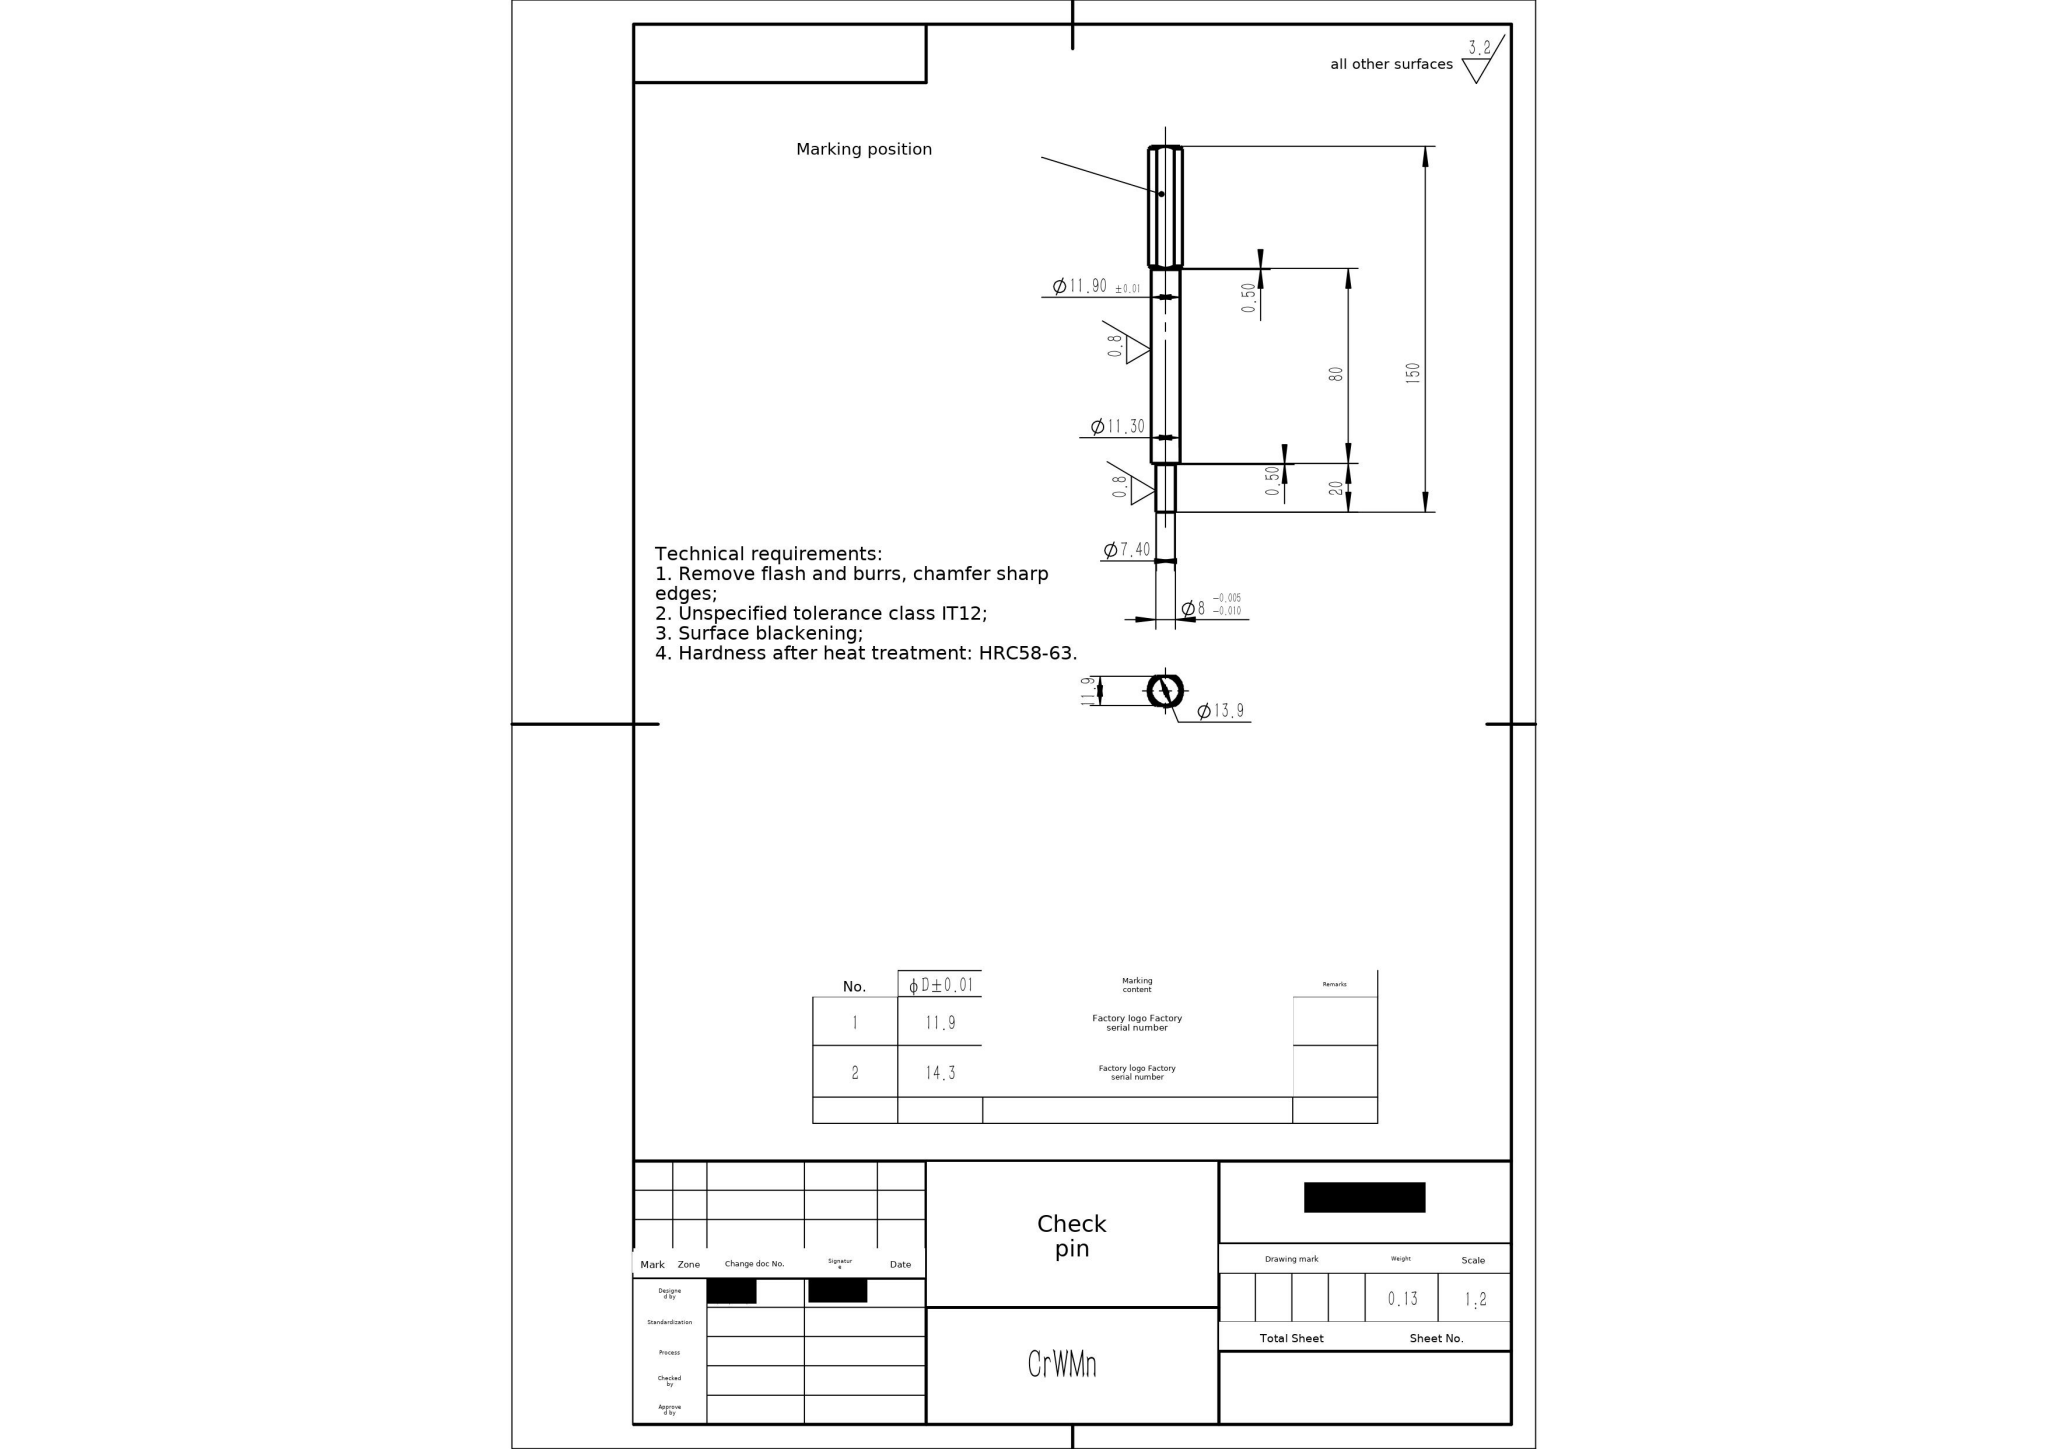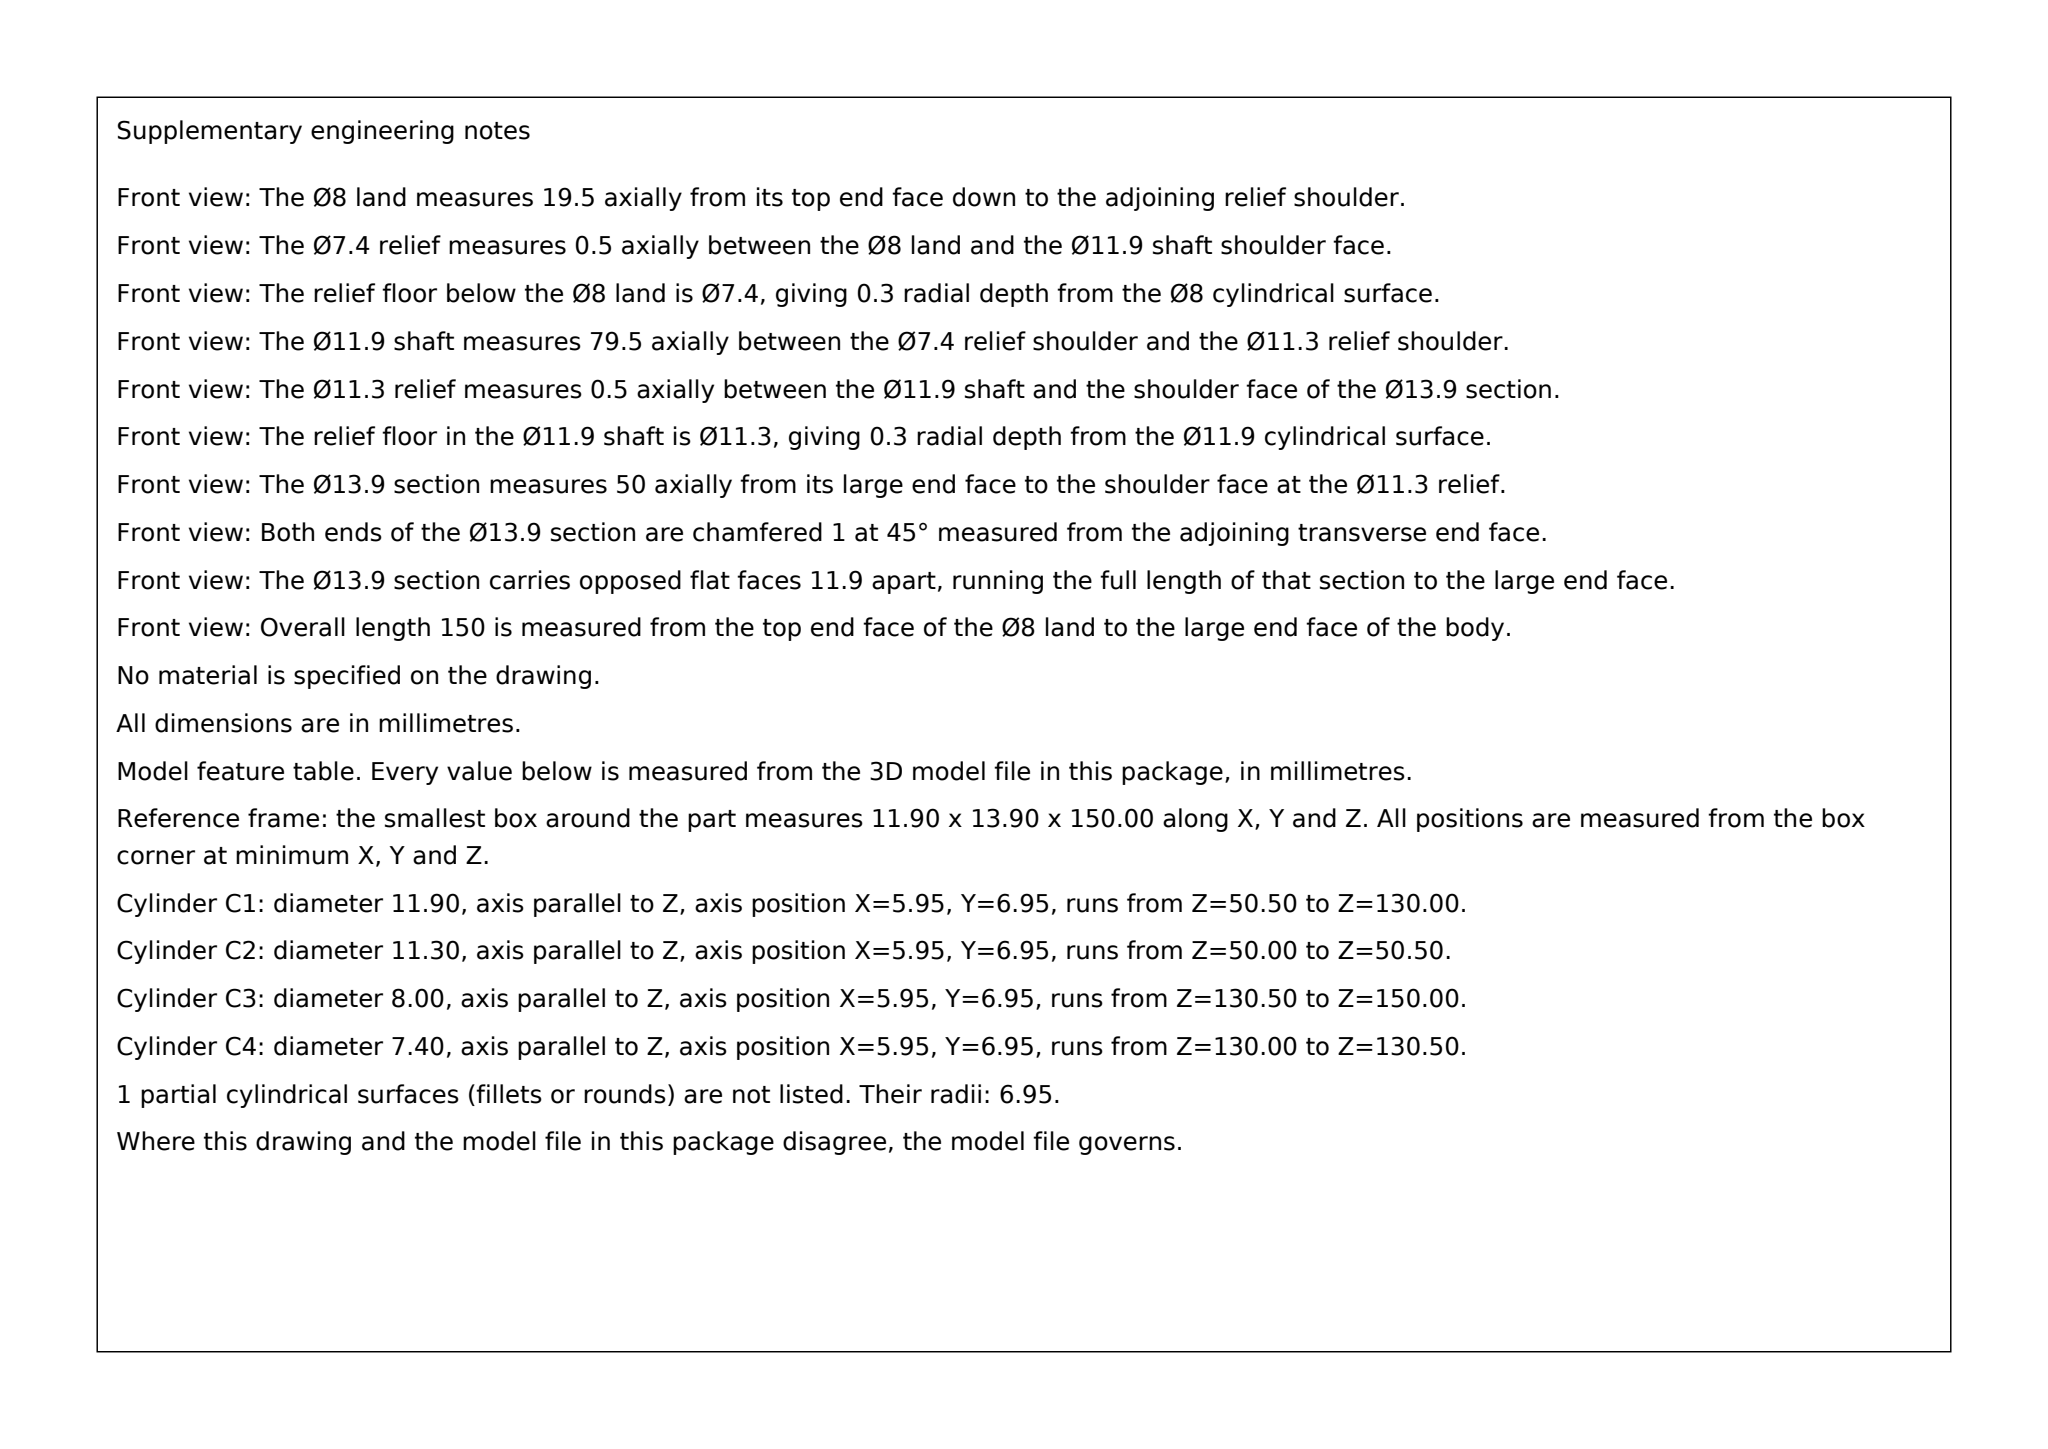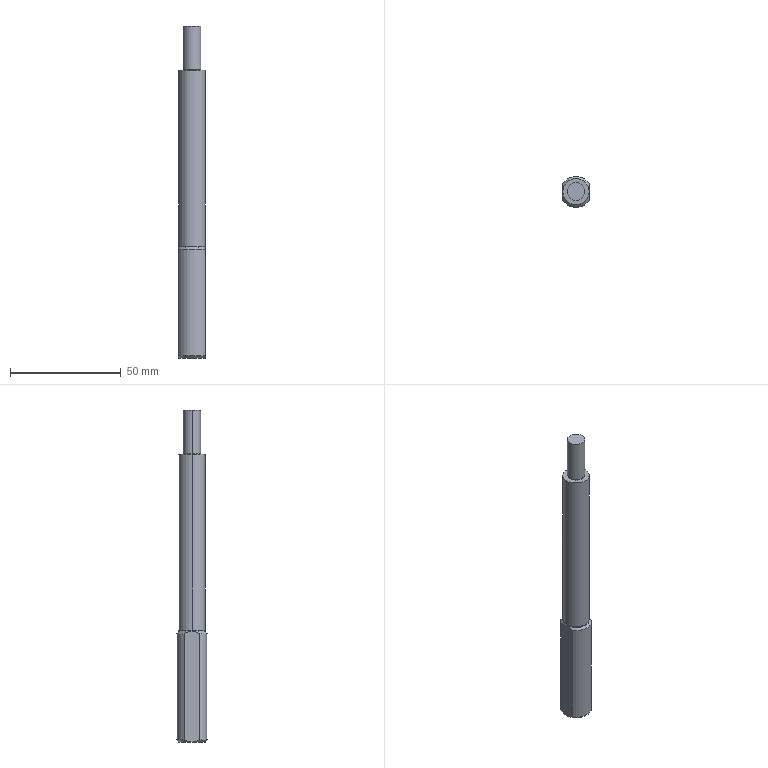Part | SolidWorks | mm | 1 solid | 22 faces | box 11.9 x 13.9 x 150 mm | volume 16965 mm3 | cylinder 10 | plane 8 | cone 4 | commonest cylinder face diameters 11.3 x2 8 x2 7.4 x2 11.9 x2 13.9 x2
Drawing notes:
2X FLAT ON Ø13.9 HEAD: 11.9 A/F x 50 LG FROM HEAD END FACE | from the solid: x-normal planes at 1.0 and 12.9 (ctr 6.95) = 11.9 across flats on Ø13.9 head; head region bounded by z-planes 0 and 50 (48 cyl + 2X C1)
45° TRANSITION BOTH ENDS Ø11.90 SHAFT, TO Ø11.30 AND TO Ø7.40 | from the solid: cones[90.0, ref_dia 11.9] count 2 at the ends of the Ø11.9 x 79.5 cylinder (z 50.5 and 130), adjoining Ø11.3 and Ø7.4 x 0.5 reliefs
STEP:
#1=CARTESIAN_POINT('',(5.65,0.,-80.));
#2=VERTEX_POINT('',#1);
#3=CARTESIAN_POINT('',(-5.65,0.,-80.));
#4=VERTEX_POINT('',#3);
#5=CARTESIAN_POINT('',(0.,0.,-80.));
#6=DIRECTION('',(0.,0.,1.));
#7=DIRECTION('',(1.,0.,0.));
#8=AXIS2_PLACEMENT_3D('',#5,#6,#7);
#9=CIRCLE('',#8,5.65);
#10=EDGE_CURVE('',#2,#4,#9,.T.);
#11=ORIENTED_EDGE('',*,*,#10,.T.);
#12=CARTESIAN_POINT('',(-5.65,0.,-79.5));
#13=VERTEX_POINT('',#12);
#14=CARTESIAN_POINT('',(-5.65,0.,20.));
#15=DIRECTION('',(0.,0.,1.));
#16=VECTOR('',#15,1000.);
#17=LINE('',#14,#16);
#18=EDGE_CURVE('',#4,#13,#17,.T.);
#19=ORIENTED_EDGE('',*,*,#18,.T.);
#20=CARTESIAN_POINT('',(5.65,0.,-79.5));
#21=VERTEX_POINT('',#20);
#22=CARTESIAN_POINT('',(0.,0.,-79.5));
#23=DIRECTION('',(0.,0.,1.));
#24=DIRECTION('',(1.,0.,0.));
#25=AXIS2_PLACEMENT_3D('',#22,#23,#24);
#26=CIRCLE('',#25,5.65);
#27=EDGE_CURVE('',#21,#13,#26,.T.);
#28=ORIENTED_EDGE('',*,*,#27,.F.);
#29=CARTESIAN_POINT('',(5.65,0.,20.));
#30=DIRECTION('',(0.,0.,1.));
#31=VECTOR('',#30,1000.);
#32=LINE('',#29,#31);
#33=EDGE_CURVE('',#2,#21,#32,.T.);
#34=ORIENTED_EDGE('',*,*,#33,.F.);
#35=EDGE_LOOP('',(#11,#19,#28,#34));
#36=FACE_OUTER_BOUND('',#35,.T.);
#37=CARTESIAN_POINT('',(0.,0.,20.));
#38=DIRECTION('',(0.,0.,1.));
#39=DIRECTION('',(1.,0.,0.));
#40=AXIS2_PLACEMENT_3D('',#37,#38,#39);
#41=CYLINDRICAL_SURFACE('',#40,5.65);
#42=ADVANCED_FACE('',(#36),#41,.T.);
#43=CARTESIAN_POINT('',(4.,0.,20.));
#44=VERTEX_POINT('',#43);
#45=CARTESIAN_POINT('',(-4.,0.,20.));
#46=VERTEX_POINT('',#45);
#47=CARTESIAN_POINT('',(0.,0.,20.));
#48=DIRECTION('',(0.,0.,1.));
#49=DIRECTION('',(1.,0.,0.));
#50=AXIS2_PLACEMENT_3D('',#47,#48,#49);
#51=CIRCLE('',#50,4.);
#52=EDGE_CURVE('',#44,#46,#51,.T.);
#53=ORIENTED_EDGE('',*,*,#52,.F.);
#54=CARTESIAN_POINT('',(4.,0.,0.5));
#55=VERTEX_POINT('',#54);
#56=CARTESIAN_POINT('',(4.,0.,20.));
#57=DIRECTION('',(0.,0.,-1.));
#58=VECTOR('',#57,1000.);
#59=LINE('',#56,#58);
#60=EDGE_CURVE('',#44,#55,#59,.T.);
#61=ORIENTED_EDGE('',*,*,#60,.T.);
#62=CARTESIAN_POINT('',(-4.,0.,0.5));
#63=VERTEX_POINT('',#62);
#64=CARTESIAN_POINT('',(0.,0.,0.5));
#65=DIRECTION('',(0.,0.,1.));
#66=DIRECTION('',(1.,0.,0.));
#67=AXIS2_PLACEMENT_3D('',#64,#65,#66);
#68=CIRCLE('',#67,4.);
#69=EDGE_CURVE('',#55,#63,#68,.T.);
#70=ORIENTED_EDGE('',*,*,#69,.T.);
#71=CARTESIAN_POINT('',(-4.,0.,20.));
#72=DIRECTION('',(0.,0.,-1.));
#73=VECTOR('',#72,1000.);
#74=LINE('',#71,#73);
#75=EDGE_CURVE('',#46,#63,#74,.T.);
#76=ORIENTED_EDGE('',*,*,#75,.F.);
#77=EDGE_LOOP('',(#53,#61,#70,#76));
#78=FACE_OUTER_BOUND('',#77,.T.);
#79=CARTESIAN_POINT('',(0.,0.,20.));
#80=DIRECTION('',(0.,0.,-1.));
#81=DIRECTION('',(-1.,0.,0.));
#82=AXIS2_PLACEMENT_3D('',#79,#80,#81);
#83=CYLINDRICAL_SURFACE('',#82,4.);
#84=ADVANCED_FACE('',(#78),#83,.T.);
#85=CARTESIAN_POINT('',(3.7,0.,0.));
#86=VERTEX_POINT('',#85);
#87=CARTESIAN_POINT('',(-3.7,0.,0.));
#88=VERTEX_POINT('',#87);
#89=CARTESIAN_POINT('',(0.,0.,0.));
#90=DIRECTION('',(0.,0.,1.));
#91=DIRECTION('',(1.,0.,0.));
#92=AXIS2_PLACEMENT_3D('',#89,#90,#91);
#93=CIRCLE('',#92,3.7);
#94=EDGE_CURVE('',#86,#88,#93,.T.);
#95=ORIENTED_EDGE('',*,*,#94,.T.);
#96=CARTESIAN_POINT('',(-3.7,0.,0.5));
#97=VERTEX_POINT('',#96);
#98=CARTESIAN_POINT('',(-3.7,0.,20.));
#99=DIRECTION('',(0.,0.,1.));
#100=VECTOR('',#99,1000.);
#101=LINE('',#98,#100);
#102=EDGE_CURVE('',#88,#97,#101,.T.);
#103=ORIENTED_EDGE('',*,*,#102,.T.);
#104=CARTESIAN_POINT('',(3.7,0.,0.5));
#105=VERTEX_POINT('',#104);
#106=CARTESIAN_POINT('',(0.,0.,0.5));
#107=DIRECTION('',(0.,0.,1.));
#108=DIRECTION('',(1.,0.,0.));
#109=AXIS2_PLACEMENT_3D('',#106,#107,#108);
#110=CIRCLE('',#109,3.7);
#111=EDGE_CURVE('',#105,#97,#110,.T.);
#112=ORIENTED_EDGE('',*,*,#111,.F.);
#113=CARTESIAN_POINT('',(3.7,0.,20.));
#114=DIRECTION('',(0.,0.,1.));
#115=VECTOR('',#114,1000.);
#116=LINE('',#113,#115);
#117=EDGE_CURVE('',#86,#105,#116,.T.);
#118=ORIENTED_EDGE('',*,*,#117,.F.);
#119=EDGE_LOOP('',(#95,#103,#112,#118));
#120=FACE_OUTER_BOUND('',#119,.T.);
#121=CARTESIAN_POINT('',(0.,0.,20.));
#122=DIRECTION('',(0.,0.,1.));
#123=DIRECTION('',(1.,0.,0.));
#124=AXIS2_PLACEMENT_3D('',#121,#122,#123);
#125=CYLINDRICAL_SURFACE('',#124,3.7);
#126=ADVANCED_FACE('',(#120),#125,.T.);
#127=CARTESIAN_POINT('',(5.95,0.,-79.5));
#128=VERTEX_POINT('',#127);
#129=CARTESIAN_POINT('',(-5.95,0.,-79.5));
#130=VERTEX_POINT('',#129);
#131=CARTESIAN_POINT('',(0.,0.,-79.5));
#132=DIRECTION('',(0.,0.,1.));
#133=DIRECTION('',(1.,0.,0.));
#134=AXIS2_PLACEMENT_3D('',#131,#132,#133);
#135=CIRCLE('',#134,5.95);
#136=EDGE_CURVE('',#128,#130,#135,.T.);
#137=ORIENTED_EDGE('',*,*,#136,.T.);
#138=CARTESIAN_POINT('',(-5.95,0.,0.));
#139=VERTEX_POINT('',#138);
#140=CARTESIAN_POINT('',(-5.95,0.,-80.));
#141=DIRECTION('',(0.,0.,1.));
#142=VECTOR('',#141,1000.);
#143=LINE('',#140,#142);
#144=EDGE_CURVE('',#130,#139,#143,.T.);
#145=ORIENTED_EDGE('',*,*,#144,.T.);
#146=CARTESIAN_POINT('',(5.95,0.,0.));
#147=VERTEX_POINT('',#146);
#148=CARTESIAN_POINT('',(0.,0.,0.));
#149=DIRECTION('',(0.,0.,-1.));
#150=DIRECTION('',(-1.,0.,0.));
#151=AXIS2_PLACEMENT_3D('',#148,#149,#150);
#152=CIRCLE('',#151,5.95);
#153=EDGE_CURVE('',#139,#147,#152,.T.);
#154=ORIENTED_EDGE('',*,*,#153,.T.);
#155=CARTESIAN_POINT('',(5.95,0.,-80.));
#156=DIRECTION('',(0.,0.,1.));
#157=VECTOR('',#156,1000.);
#158=LINE('',#155,#157);
#159=EDGE_CURVE('',#128,#147,#158,.T.);
#160=ORIENTED_EDGE('',*,*,#159,.F.);
#161=EDGE_LOOP('',(#137,#145,#154,#160));
#162=FACE_OUTER_BOUND('',#161,.T.);
#163=CARTESIAN_POINT('',(0.,0.,-80.));
#164=DIRECTION('',(0.,0.,1.));
#165=DIRECTION('',(1.,0.,0.));
#166=AXIS2_PLACEMENT_3D('',#163,#164,#165);
#167=CYLINDRICAL_SURFACE('',#166,5.95);
#168=ADVANCED_FACE('',(#162),#167,.T.);
#169=ORIENTED_EDGE('',*,*,#144,.F.);
#170=CARTESIAN_POINT('',(0.,0.,-79.5));
#171=DIRECTION('',(0.,0.,1.));
#172=DIRECTION('',(1.,0.,0.));
#173=AXIS2_PLACEMENT_3D('',#170,#171,#172);
#174=CIRCLE('',#173,5.95);
#175=EDGE_CURVE('',#130,#128,#174,.T.);
#176=ORIENTED_EDGE('',*,*,#175,.T.);
#177=ORIENTED_EDGE('',*,*,#159,.T.);
#178=CARTESIAN_POINT('',(0.,0.,0.));
#179=DIRECTION('',(0.,0.,-1.));
#180=DIRECTION('',(-1.,0.,0.));
#181=AXIS2_PLACEMENT_3D('',#178,#179,#180);
#182=CIRCLE('',#181,5.95);
#183=EDGE_CURVE('',#147,#139,#182,.T.);
#184=ORIENTED_EDGE('',*,*,#183,.T.);
#185=EDGE_LOOP('',(#169,#176,#177,#184));
#186=FACE_OUTER_BOUND('',#185,.T.);
#187=CARTESIAN_POINT('',(0.,0.,-80.));
#188=DIRECTION('',(0.,0.,1.));
#189=DIRECTION('',(1.,0.,0.));
#190=AXIS2_PLACEMENT_3D('',#187,#188,#189);
#191=CYLINDRICAL_SURFACE('',#190,5.95);
#192=ADVANCED_FACE('',(#186),#191,.T.);
#193=ORIENTED_EDGE('',*,*,#183,.F.);
#194=ORIENTED_EDGE('',*,*,#153,.F.);
#195=EDGE_LOOP('',(#193,#194));
#196=FACE_OUTER_BOUND('',#195,.T.);
#197=ORIENTED_EDGE('',*,*,#94,.F.);
#198=CARTESIAN_POINT('',(0.,0.,0.));
#199=DIRECTION('',(0.,0.,1.));
#200=DIRECTION('',(1.,0.,0.));
#201=AXIS2_PLACEMENT_3D('',#198,#199,#200);
#202=CIRCLE('',#201,3.7);
#203=EDGE_CURVE('',#88,#86,#202,.T.);
#204=ORIENTED_EDGE('',*,*,#203,.F.);
#205=EDGE_LOOP('',(#197,#204));
#206=FACE_BOUND('',#205,.T.);
#207=CARTESIAN_POINT('',(0.,0.,0.));
#208=DIRECTION('',(0.,0.,-1.));
#209=DIRECTION('',(-1.,0.,0.));
#210=AXIS2_PLACEMENT_3D('',#207,#208,#209);
#211=PLANE('',#210);
#212=ADVANCED_FACE('',(#196,#206),#211,.F.);
#213=ORIENTED_EDGE('',*,*,#102,.F.);
#214=ORIENTED_EDGE('',*,*,#203,.T.);
#215=ORIENTED_EDGE('',*,*,#117,.T.);
#216=CARTESIAN_POINT('',(0.,0.,0.5));
#217=DIRECTION('',(0.,0.,1.));
#218=DIRECTION('',(1.,0.,0.));
#219=AXIS2_PLACEMENT_3D('',#216,#217,#218);
#220=CIRCLE('',#219,3.7);
#221=EDGE_CURVE('',#97,#105,#220,.T.);
#222=ORIENTED_EDGE('',*,*,#221,.F.);
#223=EDGE_LOOP('',(#213,#214,#215,#222));
#224=FACE_OUTER_BOUND('',#223,.T.);
#225=CARTESIAN_POINT('',(0.,0.,20.));
#226=DIRECTION('',(0.,0.,1.));
#227=DIRECTION('',(1.,0.,0.));
#228=AXIS2_PLACEMENT_3D('',#225,#226,#227);
#229=CYLINDRICAL_SURFACE('',#228,3.7);
#230=ADVANCED_FACE('',(#224),#229,.T.);
#231=ORIENTED_EDGE('',*,*,#111,.T.);
#232=ORIENTED_EDGE('',*,*,#221,.T.);
#233=EDGE_LOOP('',(#231,#232));
#234=FACE_BOUND('',#233,.T.);
#235=CARTESIAN_POINT('',(0.,0.,0.5));
#236=DIRECTION('',(0.,0.,1.));
#237=DIRECTION('',(1.,0.,0.));
#238=AXIS2_PLACEMENT_3D('',#235,#236,#237);
#239=CIRCLE('',#238,4.);
#240=EDGE_CURVE('',#63,#55,#239,.T.);
#241=ORIENTED_EDGE('',*,*,#240,.F.);
#242=ORIENTED_EDGE('',*,*,#69,.F.);
#243=EDGE_LOOP('',(#241,#242));
#244=FACE_OUTER_BOUND('',#243,.T.);
#245=CARTESIAN_POINT('',(0.,4.,0.5));
#246=DIRECTION('',(0.,0.,-1.));
#247=DIRECTION('',(-1.,0.,0.));
#248=AXIS2_PLACEMENT_3D('',#245,#246,#247);
#249=PLANE('',#248);
#250=ADVANCED_FACE('',(#234,#244),#249,.T.);
#251=CARTESIAN_POINT('',(0.,0.,20.));
#252=DIRECTION('',(0.,0.,1.));
#253=DIRECTION('',(1.,0.,0.));
#254=AXIS2_PLACEMENT_3D('',#251,#252,#253);
#255=CIRCLE('',#254,4.);
#256=EDGE_CURVE('',#46,#44,#255,.T.);
#257=ORIENTED_EDGE('',*,*,#256,.T.);
#258=ORIENTED_EDGE('',*,*,#52,.T.);
#259=EDGE_LOOP('',(#257,#258));
#260=FACE_OUTER_BOUND('',#259,.T.);
#261=CARTESIAN_POINT('',(0.,0.,20.));
#262=DIRECTION('',(0.,0.,1.));
#263=DIRECTION('',(1.,0.,0.));
#264=AXIS2_PLACEMENT_3D('',#261,#262,#263);
#265=PLANE('',#264);
#266=ADVANCED_FACE('',(#260),#265,.T.);
#267=ORIENTED_EDGE('',*,*,#60,.F.);
#268=ORIENTED_EDGE('',*,*,#256,.F.);
#269=ORIENTED_EDGE('',*,*,#75,.T.);
#270=ORIENTED_EDGE('',*,*,#240,.T.);
#271=EDGE_LOOP('',(#267,#268,#269,#270));
#272=FACE_OUTER_BOUND('',#271,.T.);
#273=CARTESIAN_POINT('',(0.,0.,20.));
#274=DIRECTION('',(0.,0.,-1.));
#275=DIRECTION('',(-1.,0.,0.));
#276=AXIS2_PLACEMENT_3D('',#273,#274,#275);
#277=CYLINDRICAL_SURFACE('',#276,4.);
#278=ADVANCED_FACE('',(#272),#277,.T.);
#279=ORIENTED_EDGE('',*,*,#18,.F.);
#280=CARTESIAN_POINT('',(0.,0.,-80.));
#281=DIRECTION('',(0.,0.,1.));
#282=DIRECTION('',(1.,0.,0.));
#283=AXIS2_PLACEMENT_3D('',#280,#281,#282);
#284=CIRCLE('',#283,5.65);
#285=EDGE_CURVE('',#4,#2,#284,.T.);
#286=ORIENTED_EDGE('',*,*,#285,.T.);
#287=ORIENTED_EDGE('',*,*,#33,.T.);
#288=CARTESIAN_POINT('',(0.,0.,-79.5));
#289=DIRECTION('',(0.,0.,1.));
#290=DIRECTION('',(1.,0.,0.));
#291=AXIS2_PLACEMENT_3D('',#288,#289,#290);
#292=CIRCLE('',#291,5.65);
#293=EDGE_CURVE('',#13,#21,#292,.T.);
#294=ORIENTED_EDGE('',*,*,#293,.F.);
#295=EDGE_LOOP('',(#279,#286,#287,#294));
#296=FACE_OUTER_BOUND('',#295,.T.);
#297=CARTESIAN_POINT('',(0.,0.,20.));
#298=DIRECTION('',(0.,0.,1.));
#299=DIRECTION('',(1.,0.,0.));
#300=AXIS2_PLACEMENT_3D('',#297,#298,#299);
#301=CYLINDRICAL_SURFACE('',#300,5.65);
#302=ADVANCED_FACE('',(#296),#301,.T.);
#303=ORIENTED_EDGE('',*,*,#27,.T.);
#304=ORIENTED_EDGE('',*,*,#293,.T.);
#305=EDGE_LOOP('',(#303,#304));
#306=FACE_BOUND('',#305,.T.);
#307=ORIENTED_EDGE('',*,*,#136,.F.);
#308=ORIENTED_EDGE('',*,*,#175,.F.);
#309=EDGE_LOOP('',(#307,#308));
#310=FACE_OUTER_BOUND('',#309,.T.);
#311=CARTESIAN_POINT('',(0.,5.95,-79.5));
#312=DIRECTION('',(0.,0.,-1.));
#313=DIRECTION('',(-1.,0.,0.));
#314=AXIS2_PLACEMENT_3D('',#311,#312,#313);
#315=PLANE('',#314);
#316=ADVANCED_FACE('',(#306,#310),#315,.T.);
#317=CARTESIAN_POINT('',(-5.95,0.,-130.));
#318=VERTEX_POINT('',#317);
#319=CARTESIAN_POINT('',(5.95,0.,-130.));
#320=VERTEX_POINT('',#319);
#321=CARTESIAN_POINT('',(0.,0.,-130.));
#322=DIRECTION('',(0.,0.,-1.));
#323=DIRECTION('',(-1.,0.,0.));
#324=AXIS2_PLACEMENT_3D('',#321,#322,#323);
#325=CIRCLE('',#324,5.95);
#326=EDGE_CURVE('',#318,#320,#325,.T.);
#327=ORIENTED_EDGE('',*,*,#326,.T.);
#328=CARTESIAN_POINT('',(0.,0.,-130.));
#329=DIRECTION('',(0.,0.,-1.));
#330=DIRECTION('',(-1.,0.,0.));
#331=AXIS2_PLACEMENT_3D('',#328,#329,#330);
#332=CIRCLE('',#331,5.95);
#333=EDGE_CURVE('',#320,#318,#332,.T.);
#334=ORIENTED_EDGE('',*,*,#333,.T.);
#335=EDGE_LOOP('',(#327,#334));
#336=FACE_OUTER_BOUND('',#335,.T.);
#337=CARTESIAN_POINT('',(0.,0.,-130.));
#338=DIRECTION('',(0.,0.,-1.));
#339=DIRECTION('',(-1.,0.,0.));
#340=AXIS2_PLACEMENT_3D('',#337,#338,#339);
#341=PLANE('',#340);
#342=ADVANCED_FACE('',(#336),#341,.T.);
#343=CARTESIAN_POINT('',(5.95,3.592,-129.));
#344=VERTEX_POINT('',#343);
#345=CARTESIAN_POINT('',(5.95,3.592,-81.));
#346=VERTEX_POINT('',#345);
#347=CARTESIAN_POINT('',(5.95,3.592,-130.));
#348=DIRECTION('',(0.,0.,1.));
#349=VECTOR('',#348,1000.);
#350=LINE('',#347,#349);
#351=EDGE_CURVE('',#344,#346,#350,.T.);
#352=ORIENTED_EDGE('',*,*,#351,.F.);
#353=CARTESIAN_POINT('',(-5.95,3.592,-129.));
#354=VERTEX_POINT('',#353);
#355=CARTESIAN_POINT('',(0.,0.,-129.));
#356=DIRECTION('',(0.,0.,1.));
#357=DIRECTION('',(-1.,-0.,0.));
#358=AXIS2_PLACEMENT_3D('',#355,#356,#357);
#359=CIRCLE('',#358,6.95);
#360=EDGE_CURVE('',#344,#354,#359,.T.);
#361=ORIENTED_EDGE('',*,*,#360,.T.);
#362=CARTESIAN_POINT('',(-5.95,3.592,-81.));
#363=VERTEX_POINT('',#362);
#364=CARTESIAN_POINT('',(-5.95,3.592,-130.));
#365=DIRECTION('',(0.,0.,1.));
#366=VECTOR('',#365,1000.);
#367=LINE('',#364,#366);
#368=EDGE_CURVE('',#354,#363,#367,.T.);
#369=ORIENTED_EDGE('',*,*,#368,.T.);
#370=CARTESIAN_POINT('',(0.,0.,-81.));
#371=DIRECTION('',(0.,0.,-1.));
#372=DIRECTION('',(-1.,0.,0.));
#373=AXIS2_PLACEMENT_3D('',#370,#371,#372);
#374=CIRCLE('',#373,6.95);
#375=EDGE_CURVE('',#363,#346,#374,.T.);
#376=ORIENTED_EDGE('',*,*,#375,.T.);
#377=EDGE_LOOP('',(#352,#361,#369,#376));
#378=FACE_OUTER_BOUND('',#377,.T.);
#379=CARTESIAN_POINT('',(0.,0.,-130.));
#380=DIRECTION('',(0.,0.,1.));
#381=DIRECTION('',(1.,0.,0.));
#382=AXIS2_PLACEMENT_3D('',#379,#380,#381);
#383=CYLINDRICAL_SURFACE('',#382,6.95);
#384=ADVANCED_FACE('',(#378),#383,.T.);
#385=CARTESIAN_POINT('',(-5.95,-3.592,-81.));
#386=VERTEX_POINT('',#385);
#387=CARTESIAN_POINT('',(-5.95,-3.592,-129.));
#388=VERTEX_POINT('',#387);
#389=CARTESIAN_POINT('',(-5.95,-3.592,-130.));
#390=DIRECTION('',(0.,0.,-1.));
#391=VECTOR('',#390,1000.);
#392=LINE('',#389,#391);
#393=EDGE_CURVE('',#386,#388,#392,.T.);
#394=ORIENTED_EDGE('',*,*,#393,.T.);
#395=CARTESIAN_POINT('',(5.95,-3.592,-129.));
#396=VERTEX_POINT('',#395);
#397=CARTESIAN_POINT('',(0.,0.,-129.));
#398=DIRECTION('',(0.,0.,1.));
#399=DIRECTION('',(-1.,0.,0.));
#400=AXIS2_PLACEMENT_3D('',#397,#398,#399);
#401=CIRCLE('',#400,6.95);
#402=EDGE_CURVE('',#388,#396,#401,.T.);
#403=ORIENTED_EDGE('',*,*,#402,.T.);
#404=CARTESIAN_POINT('',(5.95,-3.592,-81.));
#405=VERTEX_POINT('',#404);
#406=CARTESIAN_POINT('',(5.95,-3.592,-130.));
#407=DIRECTION('',(0.,0.,-1.));
#408=VECTOR('',#407,1000.);
#409=LINE('',#406,#408);
#410=EDGE_CURVE('',#405,#396,#409,.T.);
#411=ORIENTED_EDGE('',*,*,#410,.F.);
#412=CARTESIAN_POINT('',(0.,0.,-81.));
#413=DIRECTION('',(0.,0.,-1.));
#414=DIRECTION('',(-1.,0.,0.));
#415=AXIS2_PLACEMENT_3D('',#412,#413,#414);
#416=CIRCLE('',#415,6.95);
#417=EDGE_CURVE('',#405,#386,#416,.T.);
#418=ORIENTED_EDGE('',*,*,#417,.T.);
#419=EDGE_LOOP('',(#394,#403,#411,#418));
#420=FACE_OUTER_BOUND('',#419,.T.);
#421=CARTESIAN_POINT('',(0.,0.,-130.));
#422=DIRECTION('',(0.,0.,1.));
#423=DIRECTION('',(1.,0.,0.));
#424=AXIS2_PLACEMENT_3D('',#421,#422,#423);
#425=CYLINDRICAL_SURFACE('',#424,6.95);
#426=ADVANCED_FACE('',(#420),#425,.T.);
#427=CARTESIAN_POINT('',(-5.95,3.592,-129.));
#428=CARTESIAN_POINT('',(-5.95,3.033,-129.289));
#429=CARTESIAN_POINT('',(-5.95,2.459,-129.537));
#430=CARTESIAN_POINT('',(-5.95,1.263,-129.894));
#431=CARTESIAN_POINT('',(-5.95,0.6334,-130.));
#432=CARTESIAN_POINT('',(-5.95,0.,-130.));
#433=B_SPLINE_CURVE_WITH_KNOTS('',3,(#427,#428,#429,#430,#431,#432),.UNSPECIFIED.,.F.,.F.,(4,2,4),(0.,0.00187,0.00374),.UNSPECIFIED.);
#434=EDGE_CURVE('',#354,#318,#433,.T.);
#435=ORIENTED_EDGE('',*,*,#434,.T.);
#436=CARTESIAN_POINT('',(-5.95,0.,-130.));
#437=CARTESIAN_POINT('',(-5.95,-0.6327,-130.));
#438=CARTESIAN_POINT('',(-5.95,-1.248,-129.898));
#439=CARTESIAN_POINT('',(-5.95,-2.15,-129.63));
#440=CARTESIAN_POINT('',(-5.95,-2.447,-129.522));
#441=CARTESIAN_POINT('',(-5.95,-3.027,-129.279));
#442=CARTESIAN_POINT('',(-5.95,-3.312,-129.145));
#443=CARTESIAN_POINT('',(-5.95,-3.592,-129.));
#444=B_SPLINE_CURVE_WITH_KNOTS('',3,(#436,#437,#438,#439,#440,#441,#442,#443),.UNSPECIFIED.,.F.,.F.,(4,2,2,4),(0.,0.00187,0.002805,0.00374),.UNSPECIFIED.);
#445=EDGE_CURVE('',#318,#388,#444,.T.);
#446=ORIENTED_EDGE('',*,*,#445,.T.);
#447=ORIENTED_EDGE('',*,*,#393,.F.);
#448=CARTESIAN_POINT('',(-5.95,-0.,-80.));
#449=VERTEX_POINT('',#448);
#450=CARTESIAN_POINT('',(-5.95,-3.592,-81.));
#451=CARTESIAN_POINT('',(-5.95,-3.033,-80.711));
#452=CARTESIAN_POINT('',(-5.95,-2.459,-80.463));
#453=CARTESIAN_POINT('',(-5.95,-1.263,-80.106));
#454=CARTESIAN_POINT('',(-5.95,-0.6334,-80.));
#455=CARTESIAN_POINT('',(-5.95,-0.,-80.));
#456=B_SPLINE_CURVE_WITH_KNOTS('',3,(#450,#451,#452,#453,#454,#455),.UNSPECIFIED.,.F.,.F.,(4,2,4),(0.,0.00187,0.00374),.UNSPECIFIED.);
#457=EDGE_CURVE('',#386,#449,#456,.T.);
#458=ORIENTED_EDGE('',*,*,#457,.T.);
#459=CARTESIAN_POINT('',(-5.95,-0.,-80.));
#460=CARTESIAN_POINT('',(-5.95,0.6327,-80.));
#461=CARTESIAN_POINT('',(-5.95,1.248,-80.102));
#462=CARTESIAN_POINT('',(-5.95,2.15,-80.37));
#463=CARTESIAN_POINT('',(-5.95,2.447,-80.478));
#464=CARTESIAN_POINT('',(-5.95,3.027,-80.721));
#465=CARTESIAN_POINT('',(-5.95,3.312,-80.855));
#466=CARTESIAN_POINT('',(-5.95,3.592,-81.));
#467=B_SPLINE_CURVE_WITH_KNOTS('',3,(#459,#460,#461,#462,#463,#464,#465,#466),.UNSPECIFIED.,.F.,.F.,(4,2,2,4),(0.,0.00187,0.002805,0.00374),.UNSPECIFIED.);
#468=EDGE_CURVE('',#449,#363,#467,.T.);
#469=ORIENTED_EDGE('',*,*,#468,.T.);
#470=ORIENTED_EDGE('',*,*,#368,.F.);
#471=EDGE_LOOP('',(#435,#446,#447,#458,#469,#470));
#472=FACE_OUTER_BOUND('',#471,.T.);
#473=CARTESIAN_POINT('',(-5.95,15.,-130.));
#474=DIRECTION('',(1.,0.,0.));
#475=DIRECTION('',(-0.,1.,0.));
#476=AXIS2_PLACEMENT_3D('',#473,#474,#475);
#477=PLANE('',#476);
#478=ADVANCED_FACE('',(#472),#477,.F.);
#479=ORIENTED_EDGE('',*,*,#410,.T.);
#480=CARTESIAN_POINT('',(5.95,-3.592,-129.));
#481=CARTESIAN_POINT('',(5.95,-3.033,-129.289));
#482=CARTESIAN_POINT('',(5.95,-2.459,-129.537));
#483=CARTESIAN_POINT('',(5.95,-1.263,-129.894));
#484=CARTESIAN_POINT('',(5.95,-0.6334,-130.));
#485=CARTESIAN_POINT('',(5.95,0.,-130.));
#486=B_SPLINE_CURVE_WITH_KNOTS('',3,(#480,#481,#482,#483,#484,#485),.UNSPECIFIED.,.F.,.F.,(4,2,4),(0.,0.00187,0.00374),.UNSPECIFIED.);
#487=EDGE_CURVE('',#396,#320,#486,.T.);
#488=ORIENTED_EDGE('',*,*,#487,.T.);
#489=CARTESIAN_POINT('',(5.95,0.,-130.));
#490=CARTESIAN_POINT('',(5.95,0.6327,-130.));
#491=CARTESIAN_POINT('',(5.95,1.248,-129.898));
#492=CARTESIAN_POINT('',(5.95,2.15,-129.63));
#493=CARTESIAN_POINT('',(5.95,2.447,-129.522));
#494=CARTESIAN_POINT('',(5.95,3.027,-129.279));
#495=CARTESIAN_POINT('',(5.95,3.312,-129.145));
#496=CARTESIAN_POINT('',(5.95,3.592,-129.));
#497=B_SPLINE_CURVE_WITH_KNOTS('',3,(#489,#490,#491,#492,#493,#494,#495,#496),.UNSPECIFIED.,.F.,.F.,(4,2,2,4),(0.,0.00187,0.002805,0.00374),.UNSPECIFIED.);
#498=EDGE_CURVE('',#320,#344,#497,.T.);
#499=ORIENTED_EDGE('',*,*,#498,.T.);
#500=ORIENTED_EDGE('',*,*,#351,.T.);
#501=CARTESIAN_POINT('',(5.95,-0.,-80.));
#502=VERTEX_POINT('',#501);
#503=CARTESIAN_POINT('',(5.95,3.592,-81.));
#504=CARTESIAN_POINT('',(5.95,3.033,-80.711));
#505=CARTESIAN_POINT('',(5.95,2.459,-80.463));
#506=CARTESIAN_POINT('',(5.95,1.263,-80.106));
#507=CARTESIAN_POINT('',(5.95,0.6334,-80.));
#508=CARTESIAN_POINT('',(5.95,-0.,-80.));
#509=B_SPLINE_CURVE_WITH_KNOTS('',3,(#503,#504,#505,#506,#507,#508),.UNSPECIFIED.,.F.,.F.,(4,2,4),(0.,0.00187,0.00374),.UNSPECIFIED.);
#510=EDGE_CURVE('',#346,#502,#509,.T.);
#511=ORIENTED_EDGE('',*,*,#510,.T.);
#512=CARTESIAN_POINT('',(5.95,-0.,-80.));
#513=CARTESIAN_POINT('',(5.95,-0.6327,-80.));
#514=CARTESIAN_POINT('',(5.95,-1.248,-80.102));
#515=CARTESIAN_POINT('',(5.95,-2.15,-80.37));
#516=CARTESIAN_POINT('',(5.95,-2.447,-80.478));
#517=CARTESIAN_POINT('',(5.95,-3.027,-80.721));
#518=CARTESIAN_POINT('',(5.95,-3.312,-80.855));
#519=CARTESIAN_POINT('',(5.95,-3.592,-81.));
#520=B_SPLINE_CURVE_WITH_KNOTS('',3,(#512,#513,#514,#515,#516,#517,#518,#519),.UNSPECIFIED.,.F.,.F.,(4,2,2,4),(0.,0.00187,0.002805,0.00374),.UNSPECIFIED.);
#521=EDGE_CURVE('',#502,#405,#520,.T.);
#522=ORIENTED_EDGE('',*,*,#521,.T.);
#523=EDGE_LOOP('',(#479,#488,#499,#500,#511,#522));
#524=FACE_OUTER_BOUND('',#523,.T.);
#525=CARTESIAN_POINT('',(5.95,15.,-130.));
#526=DIRECTION('',(1.,-0.,0.));
#527=DIRECTION('',(0.,1.,0.));
#528=AXIS2_PLACEMENT_3D('',#525,#526,#527);
#529=PLANE('',#528);
#530=ADVANCED_FACE('',(#524),#529,.T.);
#531=CARTESIAN_POINT('',(0.,0.,-80.));
#532=DIRECTION('',(0.,0.,1.));
#533=DIRECTION('',(-1.,0.,0.));
#534=AXIS2_PLACEMENT_3D('',#531,#532,#533);
#535=CIRCLE('',#534,5.95);
#536=EDGE_CURVE('',#502,#449,#535,.T.);
#537=ORIENTED_EDGE('',*,*,#536,.T.);
#538=CARTESIAN_POINT('',(0.,0.,-80.));
#539=DIRECTION('',(0.,0.,1.));
#540=DIRECTION('',(-1.,0.,0.));
#541=AXIS2_PLACEMENT_3D('',#538,#539,#540);
#542=CIRCLE('',#541,5.95);
#543=EDGE_CURVE('',#449,#502,#542,.T.);
#544=ORIENTED_EDGE('',*,*,#543,.T.);
#545=EDGE_LOOP('',(#537,#544));
#546=FACE_OUTER_BOUND('',#545,.T.);
#547=ORIENTED_EDGE('',*,*,#10,.F.);
#548=ORIENTED_EDGE('',*,*,#285,.F.);
#549=EDGE_LOOP('',(#547,#548));
#550=FACE_BOUND('',#549,.T.);
#551=CARTESIAN_POINT('',(0.,0.,-80.));
#552=DIRECTION('',(0.,0.,-1.));
#553=DIRECTION('',(-1.,0.,0.));
#554=AXIS2_PLACEMENT_3D('',#551,#552,#553);
#555=PLANE('',#554);
#556=ADVANCED_FACE('',(#546,#550),#555,.F.);
#557=ORIENTED_EDGE('',*,*,#487,.F.);
#558=ORIENTED_EDGE('',*,*,#402,.F.);
#559=ORIENTED_EDGE('',*,*,#445,.F.);
#560=ORIENTED_EDGE('',*,*,#333,.F.);
#561=EDGE_LOOP('',(#557,#558,#559,#560));
#562=FACE_OUTER_BOUND('',#561,.T.);
#563=CARTESIAN_POINT('',(0.,0.,-130.));
#564=DIRECTION('',(0.,0.,1.));
#565=DIRECTION('',(1.,0.,0.));
#566=AXIS2_PLACEMENT_3D('',#563,#564,#565);
#567=CONICAL_SURFACE('',#566,5.95,0.7854);
#568=ADVANCED_FACE('',(#562),#567,.T.);
#569=ORIENTED_EDGE('',*,*,#434,.F.);
#570=ORIENTED_EDGE('',*,*,#360,.F.);
#571=ORIENTED_EDGE('',*,*,#498,.F.);
#572=ORIENTED_EDGE('',*,*,#326,.F.);
#573=EDGE_LOOP('',(#569,#570,#571,#572));
#574=FACE_OUTER_BOUND('',#573,.T.);
#575=CARTESIAN_POINT('',(0.,0.,-130.));
#576=DIRECTION('',(0.,0.,1.));
#577=DIRECTION('',(1.,0.,0.));
#578=AXIS2_PLACEMENT_3D('',#575,#576,#577);
#579=CONICAL_SURFACE('',#578,5.95,0.7854);
#580=ADVANCED_FACE('',(#574),#579,.T.);
#581=ORIENTED_EDGE('',*,*,#521,.F.);
#582=ORIENTED_EDGE('',*,*,#543,.F.);
#583=ORIENTED_EDGE('',*,*,#457,.F.);
#584=ORIENTED_EDGE('',*,*,#417,.F.);
#585=EDGE_LOOP('',(#581,#582,#583,#584));
#586=FACE_OUTER_BOUND('',#585,.T.);
#587=CARTESIAN_POINT('',(0.,0.,-81.));
#588=DIRECTION('',(0.,0.,-1.));
#589=DIRECTION('',(-1.,0.,0.));
#590=AXIS2_PLACEMENT_3D('',#587,#588,#589);
#591=CONICAL_SURFACE('',#590,6.95,0.7854);
#592=ADVANCED_FACE('',(#586),#591,.T.);
#593=ORIENTED_EDGE('',*,*,#468,.F.);
#594=ORIENTED_EDGE('',*,*,#536,.F.);
#595=ORIENTED_EDGE('',*,*,#510,.F.);
#596=ORIENTED_EDGE('',*,*,#375,.F.);
#597=EDGE_LOOP('',(#593,#594,#595,#596));
#598=FACE_OUTER_BOUND('',#597,.T.);
#599=CARTESIAN_POINT('',(0.,0.,-81.));
#600=DIRECTION('',(0.,0.,-1.));
#601=DIRECTION('',(-1.,0.,0.));
#602=AXIS2_PLACEMENT_3D('',#599,#600,#601);
#603=CONICAL_SURFACE('',#602,6.95,0.7854);
#604=ADVANCED_FACE('',(#598),#603,.T.);
#605=CLOSED_SHELL('',(#42,#84,#126,#168,#192,#212,#230,#250,#266,#278,#302,#316,#342,#384,#426,#478,#530,#556,#568,#580,#592,#604));
#606=MANIFOLD_SOLID_BREP('',#605);
#607=CARTESIAN_POINT('',(0.,0.,0.));
#608=DIRECTION('',(0.,0.,1.));
#609=DIRECTION('',(1.,0.,0.));
#610=AXIS2_PLACEMENT_3D('',#607,#608,#609);
#611=(LENGTH_UNIT()NAMED_UNIT(*)SI_UNIT(.MILLI.,.METRE.));
#612=UNCERTAINTY_MEASURE_WITH_UNIT(LENGTH_MEASURE(0.00001),#611,'','');
#613=(NAMED_UNIT(*)PLANE_ANGLE_UNIT()SI_UNIT($,.RADIAN.));
#614=(NAMED_UNIT(*)SI_UNIT($,.STERADIAN.)SOLID_ANGLE_UNIT());
#615=(GEOMETRIC_REPRESENTATION_CONTEXT(3)GLOBAL_UNCERTAINTY_ASSIGNED_CONTEXT((#612))GLOBAL_UNIT_ASSIGNED_CONTEXT((#611,#613,#614))REPRESENTATION_CONTEXT('',''));
#616=ADVANCED_BREP_SHAPE_REPRESENTATION('',(#606,#610),#615);